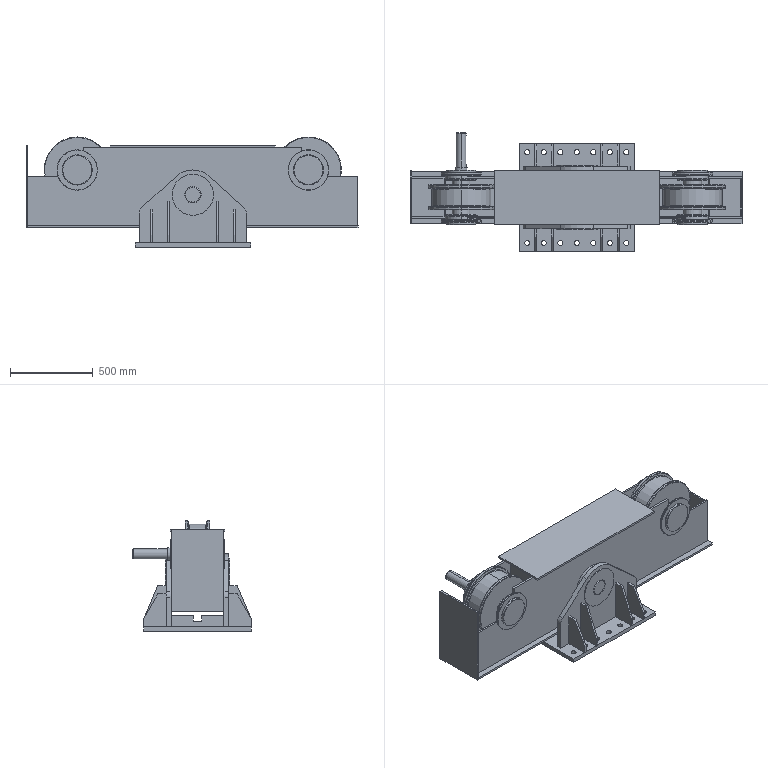Assembly | SolidWorks | mm | 35 component files | 35 solids | 470 faces | box 2010 x 716 x 667 mm | volume 111194707 mm3 | plane 225 | cylinder 141 | torus 72 | cone 32 | commonest cylinder face diameters 100 x30 31 x28 250 x16 195 x14 180 x8 245 x8 240 x8 112 x8
Bill of materials:
700X650X25 | 1 | Plain Carbon Steel | Flat rectangular plate, close to square, with two parallel rows of seven evenly spaced round through-holes along opposite edges.
Axis | 1 | Plain Carbon Steel | Solid round cylinder (pin or rod) with small chamfers or edge breaks at both ends.
BottomCover | 1 | Plain Carbon Steel | Thin, plain rectangular sheet or panel, about three times as long as it is wide, with no holes or cutouts.
Cover1 | 1 | Plain Carbon Steel | Thin, plain rectangular plate with a portrait-ratio outline (taller than wide), with no holes or cutouts.
Cover2 | 1 | Plain Carbon Steel | Plain rectangular plate, a little taller than wide, with no holes or cutouts. It looks somewhat thicker relative to its size than part-a1dd.
FlangeRib1 | 4 | Plain Carbon Steel | Flat plate with a four-sided outline: three square edges and one long angled edge cutting off one upper corner, so the top edge is shorter than the bottom edge.
FlangeRib2 | 4 | Plain Carbon Steel | Flat plate with an angled edge cutting off one corner, very similar to part-9cf3. The slope is a little steeper and the outline narrower.
RibPlate1 | 2 | Plain Carbon Steel | Plain rectangular bar or strip with an elongated outline (about 2.8:1). It is noticeably thicker relative to its width than the sheet parts.
RibPlate2 | 4 | Plain Carbon Steel | Very thin, plain rectangular sheet with a portrait-ratio outline (about 1.8:1), with no features.
SidePlate | 2 | Plain Carbon Steel | Thin, elongated flat strip with a raised center section along one long edge. Each end of that edge has a round notch near the step, and one small round through-hole sits at the center.
Support1 | 2 | Plain Carbon Steel | Flat tab with a straight bottom edge and short vertical sides. The two upper sides slope inward to a rounded top, and there is one round through-hole near the top.
Support2 | 2 | Plain Carbon Steel | Thin flat ring: a disc with a concentric circular center hole, shaped like a washer.
Support3 | 4 | Plain Carbon Steel | Thin flat annular disc (washer-like ring) with a concentric circular through-hole; plain flat faces and a cylindrical outer edge.
Support4 | 2 | Plain Carbon Steel | Flat annular disc with a concentric circular through-hole, similar to the other ring but noticeably thicker relative to its diameter.
Support5 | 1 | Plain Carbon Steel | Long rectangular prismatic bar with a single rectangular notch (slot) cut across the top face at mid-length.
TopCover | 1 | Plain Carbon Steel | Thin flat rectangular strip or plate, long and narrow, with no visible holes or cutouts.
WheelFrom | 1 | Plain Carbon Steel | Axisymmetric flanged roller or spool body: a central cylindrical drum with a raised flange at each end, short reduced-diameter necks on both sides, and stepped flanged collars at each end.
WheelMain | 1 | Plain Carbon Steel | Flanged roller body like unnamed part, plus a cylindrical shaft extending axially from one side. The shaft has an elongated slot or flat along its length.
Mates:
1. coincident | TopCover-1 face at (1250.579, 1256.349, 1665.088) dir (0, 0, 1) | SidePlate-1 face at (2250.579, 1381.349, 1665.088) dir (0, 0, -1)
2. distance | SidePlate-1 face at (1950.579, 1381.349, 2003.088) dir (0, 1, 0) | TopCover-1 face at (250.579, 1416.349, 1653.088) dir (0, 1, 0)
3. coincident | TopCover-1 face at (250.579, 1416.349, 1653.088) dir (-1, 0, 0) | SidePlate-1 face at (250.579, 1381.349, 1665.088) dir (-1, 0, 0)
4. coincident | TopCover-1 face at (250.579, 1416.349, 1653.088) dir (-1, 0, 0) | Cover1-1 face at (250.579, 1256.349, 1903.088) dir (1, 0, 0)
5. coincident | TopCover-1 face at (1250.579, 1256.349, 1653.088) dir (0, 0, -1) | Cover1-1 face at (240.579, 1096.349, 1653.088) dir (0, 0, -1)
6. coincident | TopCover-1 face at (250.579, 1096.349, 1653.088) dir (0, -1, 0) | Cover1-1 face at (240.579, 1096.349, 2153.088) dir (0, -1, 0)
7. coincident | TopCover-1 face at (2250.579, 1416.349, 1653.088) dir (1, 0, 0) | Cover2-1 face at (2250.579, 1256.349, 1809.088) dir (1, 0, 0)
8. coincident | TopCover-1 face at (1250.579, 1256.349, 1665.088) dir (0, 0, 1) | Cover2-1 face at (2250.579, 1143.349, 1665.088) dir (0, 0, -1)
9. coincident | SidePlate-2 face at (1950.579, 1143.349, 2003.088) dir (0, 1, 0) | Cover2-1 face at (2250.579, 1143.349, 1665.088) dir (0, -1, 0)
10. coincident | TopCover-1 face at (1250.579, 1256.349, 1665.088) dir (0, 0, 1) | RibPlate1-1 face at (446.579, 1143.349, 1665.088) dir (0, 0, -1)
11. coincident | SidePlate-1 face at (1950.579, 1369.349, 2003.088) dir (0, -1, 0) | RibPlate1-1 face at (446.579, 1369.349, 1745.088) dir (0, 1, 0)
12. distance | RibPlate1-1 face at (446.579, 1248.002, 1584.123) dir (-1, 0, 0) | Cover1-1 face at (250.579, 1256.349, 1903.088) dir (1, 0, 0)
13. coincident | TopCover-1 face at (1250.579, 1256.349, 1665.088) dir (0, 0, 1) | RibPlate2-1 face at (800.579, 1143.349, 1665.088) dir (0, 0, -1)
14. coincident | SidePlate-1 face at (1950.579, 1369.349, 2003.088) dir (0, -1, 0) | RibPlate2-1 face at (800.579, 1369.349, 1665.088) dir (0, 1, 0)
15. distance | RibPlate2-1 face at (800.579, 1256.349, 1903.088) dir (-1, 0, 0) | Cover1-1 face at (250.579, 1256.349, 1903.088) dir (1, 0, 0)
16. distance | RibPlate2-2 face at (1100.579, 1256.349, 1903.088) dir (-1, 0, 0) | RibPlate2-1 face at (806.579, 1256.349, 1903.088) dir (1, 0, 0)
17. coincident | TopCover-1 face at (1250.579, 1256.349, 1665.088) dir (0, 0, 1) | RibPlate2-2 face at (1100.579, 1143.349, 1665.088) dir (0, 0, -1)
18. coincident | SidePlate-1 face at (1950.579, 1369.349, 2003.088) dir (0, -1, 0) | RibPlate2-2 face at (1100.579, 1369.349, 1665.088) dir (0, 1, 0)
19. coincident | SidePlate-1 face at (1910.579, 1381.349, 2141.088) dir (0, 0, 1) | BottomCover-1 face at (1250.579, 1256.349, 2141.088) dir (0, 0, -1)
20. distance | BottomCover-1 face at (750.579, 1421.349, 2141.088) dir (0, 1, 0) | SidePlate-1 face at (1950.579, 1381.349, 2003.088) dir (0, 1, 0)
21. coincident | BottomCover-1 edge at (1250.579, 1421.349, 2141.088) dir (1, 0, 0) | assembly plane at (1250.579, 0, 0) dir (1, 0, 0)
22. coincident | SidePlate-1 face at (1950.579, 1381.349, 2003.088) dir (0, 1, 0) | Support4-1 face at (1250.579, 1381.349, 1853.088) dir (0, -1, 0)
23. concentric | SidePlate-1 face at (1250.579, 1381.349, 1853.088) dir (0, -1, 0) r 50 | Support4-1 face at (1250.579, 1399.349, 1853.088) dir (0, -1, 0) r 50
24. coincident | SidePlate-2 face at (1950.579, 1131.349, 2003.088) dir (0, -1, 0) | Support4-2 face at (1250.579, 1131.349, 1853.088) dir (0, 1, 0)
25. concentric | SidePlate-2 face at (1250.579, 1143.349, 1853.088) dir (0, -1, 0) r 50 | Support4-2 face at (1250.579, 1131.349, 1853.088) dir (0, -1, 0) r 50
26. coincident | SidePlate-2 face at (1950.579, 1143.349, 2003.088) dir (0, 1, 0) | Support3-1 face at (1250.579, 1143.349, 1853.088) dir (0, -1, 0)
27. concentric | SidePlate-2 face at (1250.579, 1143.349, 1853.088) dir (0, -1, 0) r 50 | Support3-1 face at (1250.579, 1143.349, 1853.088) dir (0, 1, 0) r 50
28. coincident | SidePlate-1 face at (1950.579, 1369.349, 2003.088) dir (0, -1, 0) | Support3-2 face at (1250.579, 1369.349, 1853.088) dir (0, 1, 0)
29. concentric | SidePlate-1 face at (1250.579, 1381.349, 1853.088) dir (0, -1, 0) r 50 | Support3-2 face at (1250.579, 1359.349, 1853.088) dir (0, 1, 0) r 50
30. coincident | TopCover-1 face at (250.579, 1096.349, 1653.088) dir (0, -1, 0) | Support1-1 face at (975.579, 1096.349, 1738.916) dir (0, 1, 0)
31. concentric | SidePlate-2 face at (1250.579, 1143.349, 1853.088) dir (0, -1, 0) r 50 | Support1-1 face at (1250.579, 1066.349, 1853.088) dir (0, 1, 0) r 50
32. parallel | TopCover-1 face at (1250.579, 1256.349, 1653.088) dir (0, 0, -1) | Support1-1 face at (925.579, 1066.349, 1561.088) dir (0, 0, -1)
33. coincident | Support1-1 face at (975.579, 1096.349, 1738.916) dir (0, 1, 0) | Support3-3 face at (1250.579, 1096.349, 1853.088) dir (0, -1, 0)
34. concentric | Support1-1 face at (1250.579, 1066.349, 1853.088) dir (0, 1, 0) r 50 | Support3-3 face at (1250.579, 1096.349, 1853.088) dir (0, 1, 0) r 50
35. coincident | Support1-1 face at (975.579, 1066.349, 1738.916) dir (0, -1, 0) | Support2-1 face at (1250.579, 1066.349, 1853.088) dir (0, 1, 0)
36. concentric | Support1-1 face at (1250.579, 1066.349, 1853.088) dir (0, 1, 0) r 50 | Support2-1 face at (1250.579, 1061.349, 1853.088) dir (0, 1, 0) r 50
37. coincident | Support1-2 face at (925.579, 1416.349, 1561.088) dir (0, 0, -1) | 700X650X25-1 face at (1250.579, 1256.349, 1561.088) dir (0, 0, 1)
38. distance | Support1-1 face at (975.579, 1066.349, 1738.916) dir (0, -1, 0) | 700X650X25-1 face at (900.579, 931.349, 1536.088) dir (0, -1, 0)
39. distance | Support1-1 face at (925.579, 1066.349, 1561.088) dir (-1, 0, 0) | 700X650X25-1 face at (900.579, 1581.349, 1536.088) dir (-1, 0, 0)
40. coincident | 700X650X25-1 face at (1250.579, 1256.349, 1561.088) dir (0, 0, 1) | Support5-1 face at (1235.579, 1416.349, 1561.088) dir (0, 0, -1)
41. coincident | Support1-2 face at (975.579, 1416.349, 1738.916) dir (0, -1, 0) | Support5-1 face at (1235.579, 1416.349, 1561.088) dir (0, 1, 0)
42. coincident | Support5-1 edge at (1250.579, 1096.349, 1561.088) dir (1, 0, 0) | assembly plane at (1250.579, 0, 0) dir (1, 0, 0)
43. coincident | Support1-1 face at (975.579, 1066.349, 1738.916) dir (0, -1, 0) | FlangeRib1-1 face at (1506.579, 1066.349, 1561.088) dir (0, 1, 0)
44. coincident | 700X650X25-1 face at (1250.579, 1256.349, 1561.088) dir (0, 0, 1) | FlangeRib1-1 face at (1506.579, 931.349, 1561.088) dir (0, 0, -1)
45. distance | FlangeRib1-1 face at (1506.579, 931.349, 1561.088) dir (1, 0, 0) | Support1-1 face at (1575.579, 1066.349, 1561.088) dir (1, 0, 0)
46. coincident | Support1-1 face at (975.579, 1066.349, 1738.916) dir (0, -1, 0) | FlangeRib2-1 face at (1406.579, 1066.349, 1561.088) dir (0, 1, 0)
47. coincident | 700X650X25-1 face at (1250.579, 1256.349, 1561.088) dir (0, 0, 1) | FlangeRib2-1 face at (1406.579, 931.349, 1561.088) dir (0, 0, -1)
48. distance | FlangeRib2-1 face at (1406.579, 931.349, 1561.088) dir (1, 0, 0) | FlangeRib1-1 face at (1494.579, 931.349, 1561.088) dir (-1, 0, 0)
49. concentric | SidePlate-2 face at (550.579, 1143.349, 2003.088) dir (0, -1, 0) r 97.5 | WheelMain-3 face at (550.579, 1647.349, 2003.088) dir (0, 1, 0) r 97.5
50. distance | SidePlate-2 face at (1950.579, 1131.349, 2003.088) dir (0, -1, 0) | WheelMain-3 face at (550.579, 1121.349, 2123.088) dir (0, 1, 0)
51. concentric | SidePlate-1 face at (1950.579, 1381.349, 2003.088) dir (0, -1, 0) r 97.5 | WheelFrom-1 face at (1950.579, 1647.349, 2003.088) dir (0, 1, 0) r 97.5
52. distance | WheelFrom-1 face at (1830.579, 1391.349, 2003.088) dir (0, -1, 0) | SidePlate-1 face at (1950.579, 1381.349, 2003.088) dir (0, 1, 0)
53. concentric | Support1-1 face at (1250.579, 1066.349, 1853.088) dir (0, 1, 0) r 50 | Axis-1 face at (1250.579, 1451.349, 1853.088) dir (0, -1, 0) r 50
54. coincident | Support2-1 face at (1250.579, 1061.349, 1853.088) dir (0, -1, 0) | Axis-1 face at (1250.579, 1061.349, 1853.088) dir (0, -1, 0)